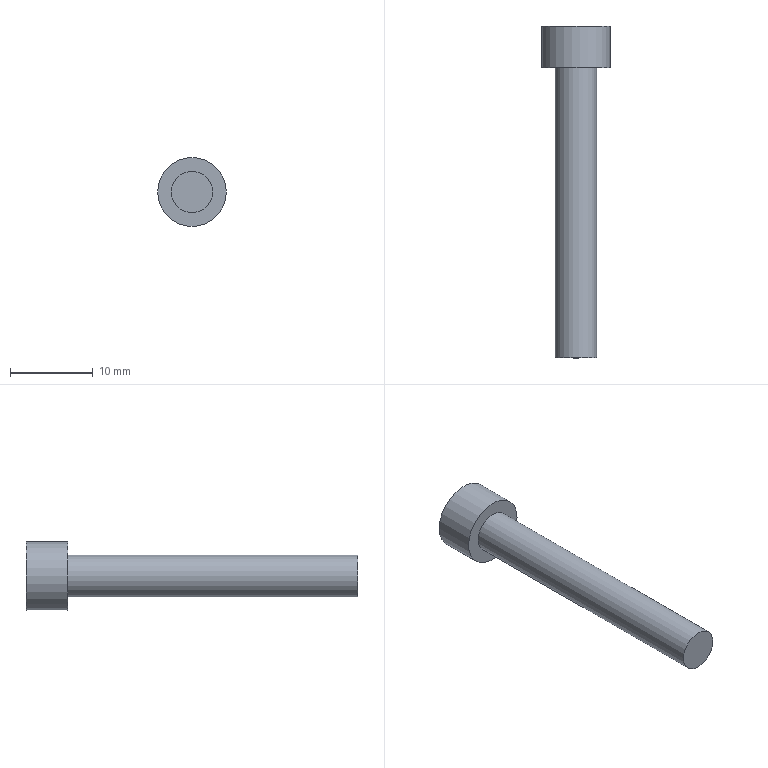Component | NX | HEX_SCREW_M5_35 | 1 solid | 12 faces | box 8.28 x 40 x 8.28 mm | volume 922 mm3 | plane 10 | cylinder 2 | commonest cylinder face diameters 8.28 x1 5 x1
STEP:
#1=CARTESIAN_POINT('',(0.,0.,0.));
#2=DIRECTION('',(0.,0.,1.));
#3=DIRECTION('',(1.,0.,0.));
#4=AXIS2_PLACEMENT_3D('',#1,#2,#3);
#5=CARTESIAN_POINT('',(-22.86,6.3,35.));
#6=VERTEX_POINT('',#5);
#7=CARTESIAN_POINT('',(-27.,6.3,35.));
#8=DIRECTION('',(0.,1.,0.));
#9=DIRECTION('',(1.,0.,0.));
#10=AXIS2_PLACEMENT_3D('',#7,#8,#9);
#11=CIRCLE('',#10,4.14);
#12=CARTESIAN_POINT('',(-27.,6.3,35.));
#13=DIRECTION('',(0.,1.,0.));
#14=DIRECTION('',(-1.,0.,0.));
#15=AXIS2_PLACEMENT_3D('',#12,#13,#14);
#16=CYLINDRICAL_SURFACE('',#15,4.14);
#17=CARTESIAN_POINT('',(3.142,0.));
#18=DIRECTION('',(1.,0.));
#19=VECTOR('',#18,1.);
#20=LINE('',#17,#19);
#21=(GEOMETRIC_REPRESENTATION_CONTEXT(2)PARAMETRIC_REPRESENTATION_CONTEXT()REPRESENTATION_CONTEXT('',''));
#22=DEFINITIONAL_REPRESENTATION('',(#20),#21);
#23=PCURVE('',#16,#22);
#24=CARTESIAN_POINT('',(-27.,6.3,35.));
#25=DIRECTION('',(0.,1.,0.));
#26=DIRECTION('',(-1.,0.,0.));
#27=AXIS2_PLACEMENT_3D('',#24,#25,#26);
#28=PLANE('',#27);
#29=CARTESIAN_POINT('',(0.,0.));
#30=DIRECTION('',(-1.,0.));
#31=AXIS2_PLACEMENT_2D('',#29,#30);
#32=CIRCLE('',#31,4.14);
#33=(GEOMETRIC_REPRESENTATION_CONTEXT(2)PARAMETRIC_REPRESENTATION_CONTEXT()REPRESENTATION_CONTEXT('',''));
#34=DEFINITIONAL_REPRESENTATION('',(#32),#33);
#35=PCURVE('',#28,#34);
#36=SURFACE_CURVE('',#11,(#23,#35),.PCURVE_S1.);
#37=EDGE_CURVE('',#6,#6,#36,.T.);
#38=ORIENTED_EDGE('',*,*,#37,.T.);
#39=CARTESIAN_POINT('',(-22.86,11.3,35.));
#40=VERTEX_POINT('',#39);
#41=CARTESIAN_POINT('',(-22.86,6.3,35.));
#42=CARTESIAN_POINT('',(-22.86,11.3,35.));
#43=B_SPLINE_CURVE_WITH_KNOTS('',1,(#41,#42),.UNSPECIFIED.,.F.,.F.,(2,2),(0.,5.),.PIECEWISE_BEZIER_KNOTS.);
#44=CARTESIAN_POINT('',(9.425,0.));
#45=DIRECTION('',(0.,1.));
#46=VECTOR('',#45,1.);
#47=LINE('',#44,#46);
#48=(GEOMETRIC_REPRESENTATION_CONTEXT(2)PARAMETRIC_REPRESENTATION_CONTEXT()REPRESENTATION_CONTEXT('',''));
#49=DEFINITIONAL_REPRESENTATION('',(#47),#48);
#50=PCURVE('',#16,#49);
#51=CARTESIAN_POINT('',(3.142,0.));
#52=DIRECTION('',(0.,1.));
#53=VECTOR('',#52,1.);
#54=LINE('',#51,#53);
#55=(GEOMETRIC_REPRESENTATION_CONTEXT(2)PARAMETRIC_REPRESENTATION_CONTEXT()REPRESENTATION_CONTEXT('',''));
#56=DEFINITIONAL_REPRESENTATION('',(#54),#55);
#57=PCURVE('',#16,#56);
#58=SEAM_CURVE('',#43,(#50,#57),.PCURVE_S1.);
#59=EDGE_CURVE('',#6,#40,#58,.T.);
#60=ORIENTED_EDGE('',*,*,#59,.T.);
#61=CARTESIAN_POINT('',(-27.,11.3,35.));
#62=DIRECTION('',(0.,1.,0.));
#63=DIRECTION('',(1.,0.,0.));
#64=AXIS2_PLACEMENT_3D('',#61,#62,#63);
#65=CIRCLE('',#64,4.14);
#66=CARTESIAN_POINT('',(3.142,5.));
#67=DIRECTION('',(1.,0.));
#68=VECTOR('',#67,1.);
#69=LINE('',#66,#68);
#70=(GEOMETRIC_REPRESENTATION_CONTEXT(2)PARAMETRIC_REPRESENTATION_CONTEXT()REPRESENTATION_CONTEXT('',''));
#71=DEFINITIONAL_REPRESENTATION('',(#69),#70);
#72=PCURVE('',#16,#71);
#73=CARTESIAN_POINT('',(-27.,11.3,35.));
#74=DIRECTION('',(0.,1.,0.));
#75=DIRECTION('',(-1.,0.,0.));
#76=AXIS2_PLACEMENT_3D('',#73,#74,#75);
#77=PLANE('',#76);
#78=CARTESIAN_POINT('',(0.,0.));
#79=DIRECTION('',(-1.,0.));
#80=AXIS2_PLACEMENT_2D('',#78,#79);
#81=CIRCLE('',#80,4.14);
#82=(GEOMETRIC_REPRESENTATION_CONTEXT(2)PARAMETRIC_REPRESENTATION_CONTEXT()REPRESENTATION_CONTEXT('',''));
#83=DEFINITIONAL_REPRESENTATION('',(#81),#82);
#84=PCURVE('',#77,#83);
#85=SURFACE_CURVE('',#65,(#72,#84),.PCURVE_S1.);
#86=EDGE_CURVE('',#40,#40,#85,.T.);
#87=ORIENTED_EDGE('',*,*,#86,.F.);
#88=ORIENTED_EDGE('',*,*,#59,.F.);
#89=EDGE_LOOP('',(#38,#60,#87,#88));
#90=FACE_BOUND('',#89,.T.);
#91=ADVANCED_FACE('',(#90),#16,.T.);
#92=CARTESIAN_POINT('',(-24.5,6.3,35.));
#93=VERTEX_POINT('',#92);
#94=CARTESIAN_POINT('',(-27.,6.3,35.));
#95=DIRECTION('',(0.,1.,0.));
#96=DIRECTION('',(1.,0.,0.));
#97=AXIS2_PLACEMENT_3D('',#94,#95,#96);
#98=CIRCLE('',#97,2.5);
#99=CARTESIAN_POINT('',(0.,0.));
#100=DIRECTION('',(-1.,0.));
#101=AXIS2_PLACEMENT_2D('',#99,#100);
#102=CIRCLE('',#101,2.5);
#103=(GEOMETRIC_REPRESENTATION_CONTEXT(2)PARAMETRIC_REPRESENTATION_CONTEXT()REPRESENTATION_CONTEXT('',''));
#104=DEFINITIONAL_REPRESENTATION('',(#102),#103);
#105=PCURVE('',#28,#104);
#106=CARTESIAN_POINT('',(-27.,-28.7,35.));
#107=DIRECTION('',(0.,1.,0.));
#108=DIRECTION('',(-1.,0.,0.));
#109=AXIS2_PLACEMENT_3D('',#106,#107,#108);
#110=CYLINDRICAL_SURFACE('',#109,2.5);
#111=CARTESIAN_POINT('',(3.142,35.));
#112=DIRECTION('',(1.,0.));
#113=VECTOR('',#112,1.);
#114=LINE('',#111,#113);
#115=(GEOMETRIC_REPRESENTATION_CONTEXT(2)PARAMETRIC_REPRESENTATION_CONTEXT()REPRESENTATION_CONTEXT('',''));
#116=DEFINITIONAL_REPRESENTATION('',(#114),#115);
#117=PCURVE('',#110,#116);
#118=SURFACE_CURVE('',#98,(#105,#117),.PCURVE_S1.);
#119=EDGE_CURVE('',#93,#93,#118,.T.);
#120=ORIENTED_EDGE('',*,*,#119,.T.);
#121=EDGE_LOOP('',(#120));
#122=FACE_BOUND('',#121,.T.);
#123=ORIENTED_EDGE('',*,*,#37,.F.);
#124=EDGE_LOOP('',(#123));
#125=FACE_BOUND('',#124,.T.);
#126=ADVANCED_FACE('',(#122,#125),#28,.F.);
#127=CARTESIAN_POINT('',(-25.,11.3,36.155));
#128=VERTEX_POINT('',#127);
#129=CARTESIAN_POINT('',(-25.,11.3,33.845));
#130=VERTEX_POINT('',#129);
#131=CARTESIAN_POINT('',(-25.,11.3,36.155));
#132=DIRECTION('',(0.,0.,-1.));
#133=VECTOR('',#132,1.);
#134=LINE('',#131,#133);
#135=CARTESIAN_POINT('',(-2.,1.155));
#136=DIRECTION('',(0.,-1.));
#137=VECTOR('',#136,1.);
#138=LINE('',#135,#137);
#139=(GEOMETRIC_REPRESENTATION_CONTEXT(2)PARAMETRIC_REPRESENTATION_CONTEXT()REPRESENTATION_CONTEXT('',''));
#140=DEFINITIONAL_REPRESENTATION('',(#138),#139);
#141=PCURVE('',#77,#140);
#142=CARTESIAN_POINT('',(-25.,8.8,36.155));
#143=DIRECTION('',(1.,0.,0.));
#144=DIRECTION('',(0.,1.,0.));
#145=AXIS2_PLACEMENT_3D('',#142,#143,#144);
#146=PLANE('',#145);
#147=CARTESIAN_POINT('',(2.5,0.));
#148=DIRECTION('',(0.,-1.));
#149=VECTOR('',#148,1.);
#150=LINE('',#147,#149);
#151=(GEOMETRIC_REPRESENTATION_CONTEXT(2)PARAMETRIC_REPRESENTATION_CONTEXT()REPRESENTATION_CONTEXT('',''));
#152=DEFINITIONAL_REPRESENTATION('',(#150),#151);
#153=PCURVE('',#146,#152);
#154=SURFACE_CURVE('',#134,(#141,#153),.PCURVE_S1.);
#155=EDGE_CURVE('',#128,#130,#154,.T.);
#156=ORIENTED_EDGE('',*,*,#155,.F.);
#157=CARTESIAN_POINT('',(-27.,11.3,37.309));
#158=VERTEX_POINT('',#157);
#159=CARTESIAN_POINT('',(-27.,11.3,37.309));
#160=DIRECTION('',(0.866,0.,-0.5));
#161=VECTOR('',#160,1.);
#162=LINE('',#159,#161);
#163=CARTESIAN_POINT('',(0.,2.309));
#164=DIRECTION('',(-0.866,-0.5));
#165=VECTOR('',#164,1.);
#166=LINE('',#163,#165);
#167=(GEOMETRIC_REPRESENTATION_CONTEXT(2)PARAMETRIC_REPRESENTATION_CONTEXT()REPRESENTATION_CONTEXT('',''));
#168=DEFINITIONAL_REPRESENTATION('',(#166),#167);
#169=PCURVE('',#77,#168);
#170=CARTESIAN_POINT('',(-27.,8.8,37.309));
#171=DIRECTION('',(0.5,0.,0.866));
#172=DIRECTION('',(-0.866,0.,0.5));
#173=AXIS2_PLACEMENT_3D('',#170,#171,#172);
#174=PLANE('',#173);
#175=CARTESIAN_POINT('',(0.,-2.5));
#176=DIRECTION('',(-1.,0.));
#177=VECTOR('',#176,1.);
#178=LINE('',#175,#177);
#179=(GEOMETRIC_REPRESENTATION_CONTEXT(2)PARAMETRIC_REPRESENTATION_CONTEXT()REPRESENTATION_CONTEXT('',''));
#180=DEFINITIONAL_REPRESENTATION('',(#178),#179);
#181=PCURVE('',#174,#180);
#182=SURFACE_CURVE('',#162,(#169,#181),.PCURVE_S1.);
#183=EDGE_CURVE('',#158,#128,#182,.T.);
#184=ORIENTED_EDGE('',*,*,#183,.F.);
#185=CARTESIAN_POINT('',(-29.,11.3,36.155));
#186=VERTEX_POINT('',#185);
#187=CARTESIAN_POINT('',(-29.,11.3,36.155));
#188=DIRECTION('',(0.866,0.,0.5));
#189=VECTOR('',#188,1.);
#190=LINE('',#187,#189);
#191=CARTESIAN_POINT('',(2.,1.155));
#192=DIRECTION('',(-0.866,0.5));
#193=VECTOR('',#192,1.);
#194=LINE('',#191,#193);
#195=(GEOMETRIC_REPRESENTATION_CONTEXT(2)PARAMETRIC_REPRESENTATION_CONTEXT()REPRESENTATION_CONTEXT('',''));
#196=DEFINITIONAL_REPRESENTATION('',(#194),#195);
#197=PCURVE('',#77,#196);
#198=CARTESIAN_POINT('',(-29.,8.8,36.155));
#199=DIRECTION('',(-0.5,0.,0.866));
#200=DIRECTION('',(-0.866,0.,-0.5));
#201=AXIS2_PLACEMENT_3D('',#198,#199,#200);
#202=PLANE('',#201);
#203=CARTESIAN_POINT('',(0.,-2.5));
#204=DIRECTION('',(-1.,0.));
#205=VECTOR('',#204,1.);
#206=LINE('',#203,#205);
#207=(GEOMETRIC_REPRESENTATION_CONTEXT(2)PARAMETRIC_REPRESENTATION_CONTEXT()REPRESENTATION_CONTEXT('',''));
#208=DEFINITIONAL_REPRESENTATION('',(#206),#207);
#209=PCURVE('',#202,#208);
#210=SURFACE_CURVE('',#190,(#197,#209),.PCURVE_S1.);
#211=EDGE_CURVE('',#186,#158,#210,.T.);
#212=ORIENTED_EDGE('',*,*,#211,.F.);
#213=CARTESIAN_POINT('',(-29.,11.3,33.845));
#214=VERTEX_POINT('',#213);
#215=CARTESIAN_POINT('',(-29.,11.3,33.845));
#216=DIRECTION('',(0.,0.,1.));
#217=VECTOR('',#216,1.);
#218=LINE('',#215,#217);
#219=CARTESIAN_POINT('',(2.,-1.155));
#220=DIRECTION('',(0.,1.));
#221=VECTOR('',#220,1.);
#222=LINE('',#219,#221);
#223=(GEOMETRIC_REPRESENTATION_CONTEXT(2)PARAMETRIC_REPRESENTATION_CONTEXT()REPRESENTATION_CONTEXT('',''));
#224=DEFINITIONAL_REPRESENTATION('',(#222),#223);
#225=PCURVE('',#77,#224);
#226=CARTESIAN_POINT('',(-29.,8.8,33.845));
#227=DIRECTION('',(-1.,0.,0.));
#228=DIRECTION('',(0.,-1.,0.));
#229=AXIS2_PLACEMENT_3D('',#226,#227,#228);
#230=PLANE('',#229);
#231=CARTESIAN_POINT('',(-2.5,0.));
#232=DIRECTION('',(0.,1.));
#233=VECTOR('',#232,1.);
#234=LINE('',#231,#233);
#235=(GEOMETRIC_REPRESENTATION_CONTEXT(2)PARAMETRIC_REPRESENTATION_CONTEXT()REPRESENTATION_CONTEXT('',''));
#236=DEFINITIONAL_REPRESENTATION('',(#234),#235);
#237=PCURVE('',#230,#236);
#238=SURFACE_CURVE('',#218,(#225,#237),.PCURVE_S1.);
#239=EDGE_CURVE('',#214,#186,#238,.T.);
#240=ORIENTED_EDGE('',*,*,#239,.F.);
#241=CARTESIAN_POINT('',(-27.,11.3,32.691));
#242=VERTEX_POINT('',#241);
#243=CARTESIAN_POINT('',(-27.,11.3,32.691));
#244=DIRECTION('',(-0.866,0.,0.5));
#245=VECTOR('',#244,1.);
#246=LINE('',#243,#245);
#247=CARTESIAN_POINT('',(0.,-2.309));
#248=DIRECTION('',(0.866,0.5));
#249=VECTOR('',#248,1.);
#250=LINE('',#247,#249);
#251=(GEOMETRIC_REPRESENTATION_CONTEXT(2)PARAMETRIC_REPRESENTATION_CONTEXT()REPRESENTATION_CONTEXT('',''));
#252=DEFINITIONAL_REPRESENTATION('',(#250),#251);
#253=PCURVE('',#77,#252);
#254=CARTESIAN_POINT('',(-27.,8.8,32.691));
#255=DIRECTION('',(-0.5,0.,-0.866));
#256=DIRECTION('',(0.866,0.,-0.5));
#257=AXIS2_PLACEMENT_3D('',#254,#255,#256);
#258=PLANE('',#257);
#259=CARTESIAN_POINT('',(0.,-2.5));
#260=DIRECTION('',(-1.,0.));
#261=VECTOR('',#260,1.);
#262=LINE('',#259,#261);
#263=(GEOMETRIC_REPRESENTATION_CONTEXT(2)PARAMETRIC_REPRESENTATION_CONTEXT()REPRESENTATION_CONTEXT('',''));
#264=DEFINITIONAL_REPRESENTATION('',(#262),#263);
#265=PCURVE('',#258,#264);
#266=SURFACE_CURVE('',#246,(#253,#265),.PCURVE_S1.);
#267=EDGE_CURVE('',#242,#214,#266,.T.);
#268=ORIENTED_EDGE('',*,*,#267,.F.);
#269=CARTESIAN_POINT('',(-25.,11.3,33.845));
#270=DIRECTION('',(-0.866,0.,-0.5));
#271=VECTOR('',#270,1.);
#272=LINE('',#269,#271);
#273=CARTESIAN_POINT('',(-2.,-1.155));
#274=DIRECTION('',(0.866,-0.5));
#275=VECTOR('',#274,1.);
#276=LINE('',#273,#275);
#277=(GEOMETRIC_REPRESENTATION_CONTEXT(2)PARAMETRIC_REPRESENTATION_CONTEXT()REPRESENTATION_CONTEXT('',''));
#278=DEFINITIONAL_REPRESENTATION('',(#276),#277);
#279=PCURVE('',#77,#278);
#280=CARTESIAN_POINT('',(-25.,8.8,33.845));
#281=DIRECTION('',(0.5,0.,-0.866));
#282=DIRECTION('',(0.866,0.,0.5));
#283=AXIS2_PLACEMENT_3D('',#280,#281,#282);
#284=PLANE('',#283);
#285=CARTESIAN_POINT('',(0.,-2.5));
#286=DIRECTION('',(-1.,0.));
#287=VECTOR('',#286,1.);
#288=LINE('',#285,#287);
#289=(GEOMETRIC_REPRESENTATION_CONTEXT(2)PARAMETRIC_REPRESENTATION_CONTEXT()REPRESENTATION_CONTEXT('',''));
#290=DEFINITIONAL_REPRESENTATION('',(#288),#289);
#291=PCURVE('',#284,#290);
#292=SURFACE_CURVE('',#272,(#279,#291),.PCURVE_S1.);
#293=EDGE_CURVE('',#130,#242,#292,.T.);
#294=ORIENTED_EDGE('',*,*,#293,.F.);
#295=EDGE_LOOP('',(#156,#184,#212,#240,#268,#294));
#296=FACE_BOUND('',#295,.T.);
#297=ORIENTED_EDGE('',*,*,#86,.T.);
#298=EDGE_LOOP('',(#297));
#299=FACE_BOUND('',#298,.T.);
#300=ADVANCED_FACE('',(#296,#299),#77,.T.);
#301=CARTESIAN_POINT('',(-24.5,-28.7,35.));
#302=VERTEX_POINT('',#301);
#303=CARTESIAN_POINT('',(-27.,-28.7,35.));
#304=DIRECTION('',(0.,1.,0.));
#305=DIRECTION('',(1.,0.,0.));
#306=AXIS2_PLACEMENT_3D('',#303,#304,#305);
#307=CIRCLE('',#306,2.5);
#308=CARTESIAN_POINT('',(3.142,0.));
#309=DIRECTION('',(1.,0.));
#310=VECTOR('',#309,1.);
#311=LINE('',#308,#310);
#312=(GEOMETRIC_REPRESENTATION_CONTEXT(2)PARAMETRIC_REPRESENTATION_CONTEXT()REPRESENTATION_CONTEXT('',''));
#313=DEFINITIONAL_REPRESENTATION('',(#311),#312);
#314=PCURVE('',#110,#313);
#315=CARTESIAN_POINT('',(-27.,-28.7,35.));
#316=DIRECTION('',(0.,1.,0.));
#317=DIRECTION('',(-1.,0.,0.));
#318=AXIS2_PLACEMENT_3D('',#315,#316,#317);
#319=PLANE('',#318);
#320=CARTESIAN_POINT('',(0.,0.));
#321=DIRECTION('',(-1.,0.));
#322=AXIS2_PLACEMENT_2D('',#320,#321);
#323=CIRCLE('',#322,2.5);
#324=(GEOMETRIC_REPRESENTATION_CONTEXT(2)PARAMETRIC_REPRESENTATION_CONTEXT()REPRESENTATION_CONTEXT('',''));
#325=DEFINITIONAL_REPRESENTATION('',(#323),#324);
#326=PCURVE('',#319,#325);
#327=SURFACE_CURVE('',#307,(#314,#326),.PCURVE_S1.);
#328=EDGE_CURVE('',#302,#302,#327,.T.);
#329=ORIENTED_EDGE('',*,*,#328,.T.);
#330=CARTESIAN_POINT('',(-24.5,-28.7,35.));
#331=CARTESIAN_POINT('',(-24.5,6.3,35.));
#332=B_SPLINE_CURVE_WITH_KNOTS('',1,(#330,#331),.UNSPECIFIED.,.F.,.F.,(2,2),(0.,35.),.PIECEWISE_BEZIER_KNOTS.);
#333=CARTESIAN_POINT('',(9.425,0.));
#334=DIRECTION('',(0.,1.));
#335=VECTOR('',#334,1.);
#336=LINE('',#333,#335);
#337=(GEOMETRIC_REPRESENTATION_CONTEXT(2)PARAMETRIC_REPRESENTATION_CONTEXT()REPRESENTATION_CONTEXT('',''));
#338=DEFINITIONAL_REPRESENTATION('',(#336),#337);
#339=PCURVE('',#110,#338);
#340=CARTESIAN_POINT('',(3.142,0.));
#341=DIRECTION('',(0.,1.));
#342=VECTOR('',#341,1.);
#343=LINE('',#340,#342);
#344=(GEOMETRIC_REPRESENTATION_CONTEXT(2)PARAMETRIC_REPRESENTATION_CONTEXT()REPRESENTATION_CONTEXT('',''));
#345=DEFINITIONAL_REPRESENTATION('',(#343),#344);
#346=PCURVE('',#110,#345);
#347=SEAM_CURVE('',#332,(#339,#346),.PCURVE_S1.);
#348=EDGE_CURVE('',#302,#93,#347,.T.);
#349=ORIENTED_EDGE('',*,*,#348,.T.);
#350=ORIENTED_EDGE('',*,*,#119,.F.);
#351=ORIENTED_EDGE('',*,*,#348,.F.);
#352=EDGE_LOOP('',(#329,#349,#350,#351));
#353=FACE_BOUND('',#352,.T.);
#354=ADVANCED_FACE('',(#353),#110,.T.);
#355=ORIENTED_EDGE('',*,*,#328,.F.);
#356=EDGE_LOOP('',(#355));
#357=FACE_BOUND('',#356,.T.);
#358=ADVANCED_FACE('',(#357),#319,.F.);
#359=ORIENTED_EDGE('',*,*,#155,.T.);
#360=CARTESIAN_POINT('',(-25.,8.8,33.845));
#361=VERTEX_POINT('',#360);
#362=CARTESIAN_POINT('',(-25.,8.8,33.845));
#363=DIRECTION('',(0.,-1.,0.));
#364=VECTOR('',#363,1.);
#365=LINE('',#362,#364);
#366=CARTESIAN_POINT('',(0.,-2.309));
#367=DIRECTION('',(-1.,0.));
#368=VECTOR('',#367,1.);
#369=LINE('',#366,#368);
#370=(GEOMETRIC_REPRESENTATION_CONTEXT(2)PARAMETRIC_REPRESENTATION_CONTEXT()REPRESENTATION_CONTEXT('',''));
#371=DEFINITIONAL_REPRESENTATION('',(#369),#370);
#372=PCURVE('',#146,#371);
#373=CARTESIAN_POINT('',(0.,0.));
#374=DIRECTION('',(0.,1.));
#375=VECTOR('',#374,1.);
#376=LINE('',#373,#375);
#377=(GEOMETRIC_REPRESENTATION_CONTEXT(2)PARAMETRIC_REPRESENTATION_CONTEXT()REPRESENTATION_CONTEXT('',''));
#378=DEFINITIONAL_REPRESENTATION('',(#376),#377);
#379=PCURVE('',#284,#378);
#380=SURFACE_CURVE('',#365,(#372,#379),.PCURVE_S1.);
#381=EDGE_CURVE('',#130,#361,#380,.T.);
#382=ORIENTED_EDGE('',*,*,#381,.T.);
#383=CARTESIAN_POINT('',(-25.,8.8,36.155));
#384=VERTEX_POINT('',#383);
#385=CARTESIAN_POINT('',(-25.,8.8,36.155));
#386=DIRECTION('',(0.,0.,1.));
#387=VECTOR('',#386,1.);
#388=LINE('',#385,#387);
#389=CARTESIAN_POINT('',(0.,0.));
#390=DIRECTION('',(0.,1.));
#391=VECTOR('',#390,1.);
#392=LINE('',#389,#391);
#393=(GEOMETRIC_REPRESENTATION_CONTEXT(2)PARAMETRIC_REPRESENTATION_CONTEXT()REPRESENTATION_CONTEXT('',''));
#394=DEFINITIONAL_REPRESENTATION('',(#392),#393);
#395=PCURVE('',#146,#394);
#396=CARTESIAN_POINT('',(-27.,8.8,35.));
#397=DIRECTION('',(0.,1.,0.));
#398=DIRECTION('',(-1.,0.,0.));
#399=AXIS2_PLACEMENT_3D('',#396,#397,#398);
#400=PLANE('',#399);
#401=CARTESIAN_POINT('',(-2.,1.155));
#402=DIRECTION('',(0.,1.));
#403=VECTOR('',#402,1.);
#404=LINE('',#401,#403);
#405=(GEOMETRIC_REPRESENTATION_CONTEXT(2)PARAMETRIC_REPRESENTATION_CONTEXT()REPRESENTATION_CONTEXT('',''));
#406=DEFINITIONAL_REPRESENTATION('',(#404),#405);
#407=PCURVE('',#400,#406);
#408=SURFACE_CURVE('',#388,(#395,#407),.PCURVE_S1.);
#409=EDGE_CURVE('',#361,#384,#408,.T.);
#410=ORIENTED_EDGE('',*,*,#409,.T.);
#411=CARTESIAN_POINT('',(-25.,8.8,36.155));
#412=DIRECTION('',(0.,-1.,0.));
#413=VECTOR('',#412,1.);
#414=LINE('',#411,#413);
#415=CARTESIAN_POINT('',(0.,0.));
#416=DIRECTION('',(-1.,0.));
#417=VECTOR('',#416,1.);
#418=LINE('',#415,#417);
#419=(GEOMETRIC_REPRESENTATION_CONTEXT(2)PARAMETRIC_REPRESENTATION_CONTEXT()REPRESENTATION_CONTEXT('',''));
#420=DEFINITIONAL_REPRESENTATION('',(#418),#419);
#421=PCURVE('',#146,#420);
#422=CARTESIAN_POINT('',(-2.309,0.));
#423=DIRECTION('',(0.,1.));
#424=VECTOR('',#423,1.);
#425=LINE('',#422,#424);
#426=(GEOMETRIC_REPRESENTATION_CONTEXT(2)PARAMETRIC_REPRESENTATION_CONTEXT()REPRESENTATION_CONTEXT('',''));
#427=DEFINITIONAL_REPRESENTATION('',(#425),#426);
#428=PCURVE('',#174,#427);
#429=SURFACE_CURVE('',#414,(#421,#428),.PCURVE_S1.);
#430=EDGE_CURVE('',#128,#384,#429,.T.);
#431=ORIENTED_EDGE('',*,*,#430,.F.);
#432=EDGE_LOOP('',(#359,#382,#410,#431));
#433=FACE_BOUND('',#432,.T.);
#434=ADVANCED_FACE('',(#433),#146,.F.);
#435=ORIENTED_EDGE('',*,*,#293,.T.);
#436=CARTESIAN_POINT('',(-27.,8.8,32.691));
#437=VERTEX_POINT('',#436);
#438=CARTESIAN_POINT('',(-27.,8.8,32.691));
#439=DIRECTION('',(0.,-1.,0.));
#440=VECTOR('',#439,1.);
#441=LINE('',#438,#440);
#442=CARTESIAN_POINT('',(-2.309,0.));
#443=DIRECTION('',(0.,1.));
#444=VECTOR('',#443,1.);
#445=LINE('',#442,#444);
#446=(GEOMETRIC_REPRESENTATION_CONTEXT(2)PARAMETRIC_REPRESENTATION_CONTEXT()REPRESENTATION_CONTEXT('',''));
#447=DEFINITIONAL_REPRESENTATION('',(#445),#446);
#448=PCURVE('',#284,#447);
#449=CARTESIAN_POINT('',(0.,0.));
#450=DIRECTION('',(0.,1.));
#451=VECTOR('',#450,1.);
#452=LINE('',#449,#451);
#453=(GEOMETRIC_REPRESENTATION_CONTEXT(2)PARAMETRIC_REPRESENTATION_CONTEXT()REPRESENTATION_CONTEXT('',''));
#454=DEFINITIONAL_REPRESENTATION('',(#452),#453);
#455=PCURVE('',#258,#454);
#456=SURFACE_CURVE('',#441,(#448,#455),.PCURVE_S1.);
#457=EDGE_CURVE('',#242,#437,#456,.T.);
#458=ORIENTED_EDGE('',*,*,#457,.T.);
#459=CARTESIAN_POINT('',(-25.,8.8,33.845));
#460=DIRECTION('',(0.866,0.,0.5));
#461=VECTOR('',#460,1.);
#462=LINE('',#459,#461);
#463=CARTESIAN_POINT('',(0.,0.));
#464=DIRECTION('',(1.,0.));
#465=VECTOR('',#464,1.);
#466=LINE('',#463,#465);
#467=(GEOMETRIC_REPRESENTATION_CONTEXT(2)PARAMETRIC_REPRESENTATION_CONTEXT()REPRESENTATION_CONTEXT('',''));
#468=DEFINITIONAL_REPRESENTATION('',(#466),#467);
#469=PCURVE('',#284,#468);
#470=CARTESIAN_POINT('',(-2.,-1.155));
#471=DIRECTION('',(-0.866,0.5));
#472=VECTOR('',#471,1.);
#473=LINE('',#470,#472);
#474=(GEOMETRIC_REPRESENTATION_CONTEXT(2)PARAMETRIC_REPRESENTATION_CONTEXT()REPRESENTATION_CONTEXT('',''));
#475=DEFINITIONAL_REPRESENTATION('',(#473),#474);
#476=PCURVE('',#400,#475);
#477=SURFACE_CURVE('',#462,(#469,#476),.PCURVE_S1.);
#478=EDGE_CURVE('',#437,#361,#477,.T.);
#479=ORIENTED_EDGE('',*,*,#478,.T.);
#480=ORIENTED_EDGE('',*,*,#381,.F.);
#481=EDGE_LOOP('',(#435,#458,#479,#480));
#482=FACE_BOUND('',#481,.T.);
#483=ADVANCED_FACE('',(#482),#284,.F.);
#484=ORIENTED_EDGE('',*,*,#267,.T.);
#485=CARTESIAN_POINT('',(-29.,8.8,33.845));
#486=VERTEX_POINT('',#485);
#487=CARTESIAN_POINT('',(-29.,8.8,33.845));
#488=DIRECTION('',(0.,-1.,0.));
#489=VECTOR('',#488,1.);
#490=LINE('',#487,#489);
#491=CARTESIAN_POINT('',(-2.309,0.));
#492=DIRECTION('',(0.,1.));
#493=VECTOR('',#492,1.);
#494=LINE('',#491,#493);
#495=(GEOMETRIC_REPRESENTATION_CONTEXT(2)PARAMETRIC_REPRESENTATION_CONTEXT()REPRESENTATION_CONTEXT('',''));
#496=DEFINITIONAL_REPRESENTATION('',(#494),#495);
#497=PCURVE('',#258,#496);
#498=CARTESIAN_POINT('',(0.,0.));
#499=DIRECTION('',(1.,0.));
#500=VECTOR('',#499,1.);
#501=LINE('',#498,#500);
#502=(GEOMETRIC_REPRESENTATION_CONTEXT(2)PARAMETRIC_REPRESENTATION_CONTEXT()REPRESENTATION_CONTEXT('',''));
#503=DEFINITIONAL_REPRESENTATION('',(#501),#502);
#504=PCURVE('',#230,#503);
#505=SURFACE_CURVE('',#490,(#497,#504),.PCURVE_S1.);
#506=EDGE_CURVE('',#214,#486,#505,.T.);
#507=ORIENTED_EDGE('',*,*,#506,.T.);
#508=CARTESIAN_POINT('',(-27.,8.8,32.691));
#509=DIRECTION('',(0.866,0.,-0.5));
#510=VECTOR('',#509,1.);
#511=LINE('',#508,#510);
#512=CARTESIAN_POINT('',(0.,0.));
#513=DIRECTION('',(1.,0.));
#514=VECTOR('',#513,1.);
#515=LINE('',#512,#514);
#516=(GEOMETRIC_REPRESENTATION_CONTEXT(2)PARAMETRIC_REPRESENTATION_CONTEXT()REPRESENTATION_CONTEXT('',''));
#517=DEFINITIONAL_REPRESENTATION('',(#515),#516);
#518=PCURVE('',#258,#517);
#519=CARTESIAN_POINT('',(0.,-2.309));
#520=DIRECTION('',(-0.866,-0.5));
#521=VECTOR('',#520,1.);
#522=LINE('',#519,#521);
#523=(GEOMETRIC_REPRESENTATION_CONTEXT(2)PARAMETRIC_REPRESENTATION_CONTEXT()REPRESENTATION_CONTEXT('',''));
#524=DEFINITIONAL_REPRESENTATION('',(#522),#523);
#525=PCURVE('',#400,#524);
#526=SURFACE_CURVE('',#511,(#518,#525),.PCURVE_S1.);
#527=EDGE_CURVE('',#486,#437,#526,.T.);
#528=ORIENTED_EDGE('',*,*,#527,.T.);
#529=ORIENTED_EDGE('',*,*,#457,.F.);
#530=EDGE_LOOP('',(#484,#507,#528,#529));
#531=FACE_BOUND('',#530,.T.);
#532=ADVANCED_FACE('',(#531),#258,.F.);
#533=ORIENTED_EDGE('',*,*,#239,.T.);
#534=CARTESIAN_POINT('',(-29.,8.8,36.155));
#535=VERTEX_POINT('',#534);
#536=CARTESIAN_POINT('',(-29.,8.8,36.155));
#537=DIRECTION('',(0.,-1.,0.));
#538=VECTOR('',#537,1.);
#539=LINE('',#536,#538);
#540=CARTESIAN_POINT('',(0.,2.309));
#541=DIRECTION('',(1.,0.));
#542=VECTOR('',#541,1.);
#543=LINE('',#540,#542);
#544=(GEOMETRIC_REPRESENTATION_CONTEXT(2)PARAMETRIC_REPRESENTATION_CONTEXT()REPRESENTATION_CONTEXT('',''));
#545=DEFINITIONAL_REPRESENTATION('',(#543),#544);
#546=PCURVE('',#230,#545);
#547=CARTESIAN_POINT('',(0.,0.));
#548=DIRECTION('',(0.,1.));
#549=VECTOR('',#548,1.);
#550=LINE('',#547,#549);
#551=(GEOMETRIC_REPRESENTATION_CONTEXT(2)PARAMETRIC_REPRESENTATION_CONTEXT()REPRESENTATION_CONTEXT('',''));
#552=DEFINITIONAL_REPRESENTATION('',(#550),#551);
#553=PCURVE('',#202,#552);
#554=SURFACE_CURVE('',#539,(#546,#553),.PCURVE_S1.);
#555=EDGE_CURVE('',#186,#535,#554,.T.);
#556=ORIENTED_EDGE('',*,*,#555,.T.);
#557=CARTESIAN_POINT('',(-29.,8.8,33.845));
#558=DIRECTION('',(0.,0.,-1.));
#559=VECTOR('',#558,1.);
#560=LINE('',#557,#559);
#561=CARTESIAN_POINT('',(0.,0.));
#562=DIRECTION('',(0.,-1.));
#563=VECTOR('',#562,1.);
#564=LINE('',#561,#563);
#565=(GEOMETRIC_REPRESENTATION_CONTEXT(2)PARAMETRIC_REPRESENTATION_CONTEXT()REPRESENTATION_CONTEXT('',''));
#566=DEFINITIONAL_REPRESENTATION('',(#564),#565);
#567=PCURVE('',#230,#566);
#568=CARTESIAN_POINT('',(2.,-1.155));
#569=DIRECTION('',(0.,-1.));
#570=VECTOR('',#569,1.);
#571=LINE('',#568,#570);
#572=(GEOMETRIC_REPRESENTATION_CONTEXT(2)PARAMETRIC_REPRESENTATION_CONTEXT()REPRESENTATION_CONTEXT('',''));
#573=DEFINITIONAL_REPRESENTATION('',(#571),#572);
#574=PCURVE('',#400,#573);
#575=SURFACE_CURVE('',#560,(#567,#574),.PCURVE_S1.);
#576=EDGE_CURVE('',#535,#486,#575,.T.);
#577=ORIENTED_EDGE('',*,*,#576,.T.);
#578=ORIENTED_EDGE('',*,*,#506,.F.);
#579=EDGE_LOOP('',(#533,#556,#577,#578));
#580=FACE_BOUND('',#579,.T.);
#581=ADVANCED_FACE('',(#580),#230,.F.);
#582=ORIENTED_EDGE('',*,*,#211,.T.);
#583=CARTESIAN_POINT('',(-27.,8.8,37.309));
#584=VERTEX_POINT('',#583);
#585=CARTESIAN_POINT('',(-27.,8.8,37.309));
#586=DIRECTION('',(0.,-1.,0.));
#587=VECTOR('',#586,1.);
#588=LINE('',#585,#587);
#589=CARTESIAN_POINT('',(-2.309,0.));
#590=DIRECTION('',(0.,1.));
#591=VECTOR('',#590,1.);
#592=LINE('',#589,#591);
#593=(GEOMETRIC_REPRESENTATION_CONTEXT(2)PARAMETRIC_REPRESENTATION_CONTEXT()REPRESENTATION_CONTEXT('',''));
#594=DEFINITIONAL_REPRESENTATION('',(#592),#593);
#595=PCURVE('',#202,#594);
#596=CARTESIAN_POINT('',(0.,0.));
#597=DIRECTION('',(0.,1.));
#598=VECTOR('',#597,1.);
#599=LINE('',#596,#598);
#600=(GEOMETRIC_REPRESENTATION_CONTEXT(2)PARAMETRIC_REPRESENTATION_CONTEXT()REPRESENTATION_CONTEXT('',''));
#601=DEFINITIONAL_REPRESENTATION('',(#599),#600);
#602=PCURVE('',#174,#601);
#603=SURFACE_CURVE('',#588,(#595,#602),.PCURVE_S1.);
#604=EDGE_CURVE('',#158,#584,#603,.T.);
#605=ORIENTED_EDGE('',*,*,#604,.T.);
#606=CARTESIAN_POINT('',(-29.,8.8,36.155));
#607=DIRECTION('',(-0.866,0.,-0.5));
#608=VECTOR('',#607,1.);
#609=LINE('',#606,#608);
#610=CARTESIAN_POINT('',(0.,0.));
#611=DIRECTION('',(1.,0.));
#612=VECTOR('',#611,1.);
#613=LINE('',#610,#612);
#614=(GEOMETRIC_REPRESENTATION_CONTEXT(2)PARAMETRIC_REPRESENTATION_CONTEXT()REPRESENTATION_CONTEXT('',''));
#615=DEFINITIONAL_REPRESENTATION('',(#613),#614);
#616=PCURVE('',#202,#615);
#617=CARTESIAN_POINT('',(2.,1.155));
#618=DIRECTION('',(0.866,-0.5));
#619=VECTOR('',#618,1.);
#620=LINE('',#617,#619);
#621=(GEOMETRIC_REPRESENTATION_CONTEXT(2)PARAMETRIC_REPRESENTATION_CONTEXT()REPRESENTATION_CONTEXT('',''));
#622=DEFINITIONAL_REPRESENTATION('',(#620),#621);
#623=PCURVE('',#400,#622);
#624=SURFACE_CURVE('',#609,(#616,#623),.PCURVE_S1.);
#625=EDGE_CURVE('',#584,#535,#624,.T.);
#626=ORIENTED_EDGE('',*,*,#625,.T.);
#627=ORIENTED_EDGE('',*,*,#555,.F.);
#628=EDGE_LOOP('',(#582,#605,#626,#627));
#629=FACE_BOUND('',#628,.T.);
#630=ADVANCED_FACE('',(#629),#202,.F.);
#631=ORIENTED_EDGE('',*,*,#183,.T.);
#632=ORIENTED_EDGE('',*,*,#430,.T.);
#633=CARTESIAN_POINT('',(-27.,8.8,37.309));
#634=DIRECTION('',(-0.866,0.,0.5));
#635=VECTOR('',#634,1.);
#636=LINE('',#633,#635);
#637=CARTESIAN_POINT('',(0.,0.));
#638=DIRECTION('',(1.,0.));
#639=VECTOR('',#638,1.);
#640=LINE('',#637,#639);
#641=(GEOMETRIC_REPRESENTATION_CONTEXT(2)PARAMETRIC_REPRESENTATION_CONTEXT()REPRESENTATION_CONTEXT('',''));
#642=DEFINITIONAL_REPRESENTATION('',(#640),#641);
#643=PCURVE('',#174,#642);
#644=CARTESIAN_POINT('',(0.,2.309));
#645=DIRECTION('',(0.866,0.5));
#646=VECTOR('',#645,1.);
#647=LINE('',#644,#646);
#648=(GEOMETRIC_REPRESENTATION_CONTEXT(2)PARAMETRIC_REPRESENTATION_CONTEXT()REPRESENTATION_CONTEXT('',''));
#649=DEFINITIONAL_REPRESENTATION('',(#647),#648);
#650=PCURVE('',#400,#649);
#651=SURFACE_CURVE('',#636,(#643,#650),.PCURVE_S1.);
#652=EDGE_CURVE('',#384,#584,#651,.T.);
#653=ORIENTED_EDGE('',*,*,#652,.T.);
#654=ORIENTED_EDGE('',*,*,#604,.F.);
#655=EDGE_LOOP('',(#631,#632,#653,#654));
#656=FACE_BOUND('',#655,.T.);
#657=ADVANCED_FACE('',(#656),#174,.F.);
#658=ORIENTED_EDGE('',*,*,#409,.F.);
#659=ORIENTED_EDGE('',*,*,#478,.F.);
#660=ORIENTED_EDGE('',*,*,#527,.F.);
#661=ORIENTED_EDGE('',*,*,#576,.F.);
#662=ORIENTED_EDGE('',*,*,#625,.F.);
#663=ORIENTED_EDGE('',*,*,#652,.F.);
#664=EDGE_LOOP('',(#658,#659,#660,#661,#662,#663));
#665=FACE_BOUND('',#664,.T.);
#666=ADVANCED_FACE('',(#665),#400,.T.);
#667=CLOSED_SHELL('',(#91,#126,#300,#354,#358,#434,#483,#532,#581,#630,#657,#666));
#668=MANIFOLD_SOLID_BREP('',#667);
#669=(LENGTH_UNIT()NAMED_UNIT(*)SI_UNIT(.MILLI.,.METRE.));
#670=UNCERTAINTY_MEASURE_WITH_UNIT(LENGTH_MEASURE(0.000002),#669,'','');
#671=(NAMED_UNIT(*)PLANE_ANGLE_UNIT()SI_UNIT($,.RADIAN.));
#672=(NAMED_UNIT(*)SI_UNIT($,.STERADIAN.)SOLID_ANGLE_UNIT());
#673=(GEOMETRIC_REPRESENTATION_CONTEXT(3)GLOBAL_UNCERTAINTY_ASSIGNED_CONTEXT((#670))GLOBAL_UNIT_ASSIGNED_CONTEXT((#669,#671,#672))REPRESENTATION_CONTEXT('',''));
#674=ADVANCED_BREP_SHAPE_REPRESENTATION('',(#4,#668),#673);